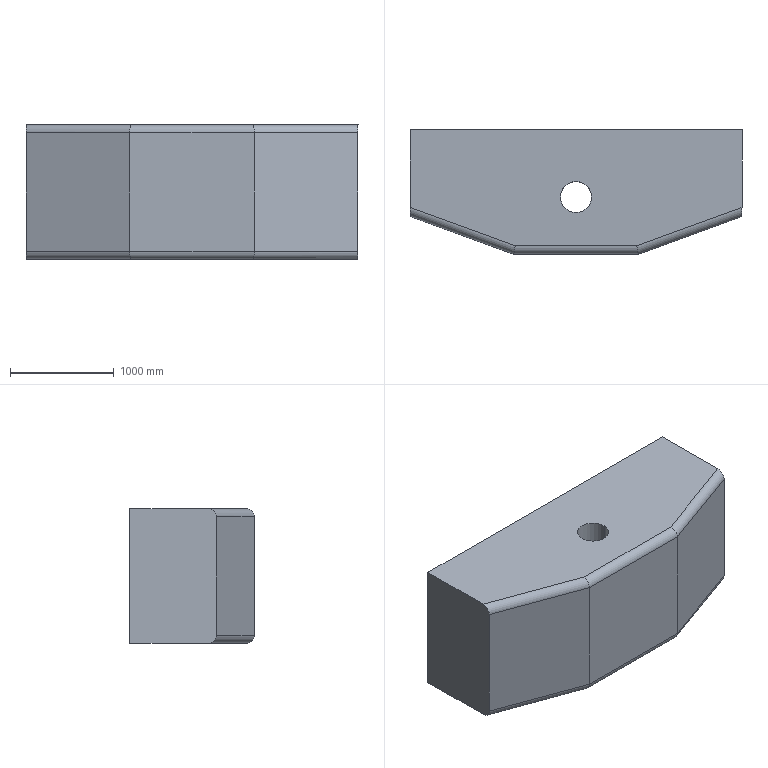Component | SolidWorks | RunningMechanism-5_7-1 | 1 solid | 16 faces | box 3200 x 1200 x 1300 mm | volume 4417803328 mm3 | cylinder 8 | plane 8 | commonest cylinder face diameters 160 x6 300 x2
build123d program:
from build123d import *

# Parameters (mm, degrees)
BOSS_EXTRUDE1_DEPTH = 650
SKETCH2_R           = 150
CUT_EXTRUDE1_DEPTH  = 2386.372
FILLET1_R           = 80


with BuildPart() as part:
    # Sketch1 → Boss-Extrude1 (new, symmetric)
    with BuildSketch(Plane.XY):
        Polygon((-1600, 0), (1600, 0), (1600, 836.03), (600, 1200), (-600, 1200), (-1600, 836.03), align=None)
    extrude(amount=BOSS_EXTRUDE1_DEPTH, both=True)

    # Sketch2 → Cut-Extrude1 (cut, through all)
    with BuildSketch(Plane.XY.offset(650)):
        with Locations((0, 650)):
            Circle(SKETCH2_R)
    extrude(amount=-CUT_EXTRUDE1_DEPTH, mode=Mode.SUBTRACT)

    # Fillet1
    fillet1_edges = [part.edges().sort_by_distance(p)[0] for p in [
        (1100, 1018.015, 650),
        (0, 1200, 650),
        (-1100, 1018.015, 650),
        (0, 1200, -650),
        (1100, 1018.015, -650),
        (-1100, 1018.015, -650),
    ]]
    fillet(fillet1_edges, radius=FILLET1_R)


solid = part.part

# Placed as in the assembly
solid = solid.moved(Location((8341.033, 54548.441, -12026.998), (180, 0, 0)))
STEP:
#1=COLOUR_RGB('',0.7922,0.8196,0.9333);
#2=FILL_AREA_STYLE_COLOUR('',#1);
#3=FILL_AREA_STYLE('',(#2));
#4=SURFACE_STYLE_FILL_AREA(#3);
#5=SURFACE_SIDE_STYLE('',(#4));
#6=SURFACE_STYLE_USAGE(.BOTH.,#5);
#7=PRESENTATION_STYLE_ASSIGNMENT((#6));
#8=CARTESIAN_POINT('',(334.293,2121.986,-499.094));
#9=VERTEX_POINT('',#8);
#10=CARTESIAN_POINT('',(322.482,2121.986,-499.094));
#11=VERTEX_POINT('',#10);
#12=CARTESIAN_POINT('',(328.387,2121.986,-499.094));
#13=DIRECTION('',(0.0000002,0.,1.));
#14=DIRECTION('',(-1.,0.,0.0000002));
#15=AXIS2_PLACEMENT_3D('',#12,#13,#14);
#16=CIRCLE('',#15,5.906);
#17=EDGE_CURVE('',#9,#11,#16,.T.);
#18=ORIENTED_EDGE('',*,*,#17,.F.);
#19=CARTESIAN_POINT('',(334.293,2121.986,-447.913));
#20=VERTEX_POINT('',#19);
#21=CARTESIAN_POINT('',(334.293,2121.986,-499.094));
#22=DIRECTION('',(0.0000002,0.,1.));
#23=VECTOR('',#22,39.37);
#24=LINE('',#21,#23);
#25=EDGE_CURVE('',#9,#20,#24,.T.);
#26=ORIENTED_EDGE('',*,*,#25,.T.);
#27=CARTESIAN_POINT('',(322.482,2121.986,-447.913));
#28=VERTEX_POINT('',#27);
#29=CARTESIAN_POINT('',(328.387,2121.986,-447.913));
#30=DIRECTION('',(0.0000002,0.,1.));
#31=DIRECTION('',(-1.,0.,0.0000002));
#32=AXIS2_PLACEMENT_3D('',#29,#30,#31);
#33=CIRCLE('',#32,5.906);
#34=EDGE_CURVE('',#20,#28,#33,.T.);
#35=ORIENTED_EDGE('',*,*,#34,.T.);
#36=CARTESIAN_POINT('',(322.482,2121.986,-499.094));
#37=DIRECTION('',(0.0000002,0.,1.));
#38=VECTOR('',#37,39.37);
#39=LINE('',#36,#38);
#40=EDGE_CURVE('',#11,#28,#39,.T.);
#41=ORIENTED_EDGE('',*,*,#40,.F.);
#42=EDGE_LOOP('',(#18,#26,#35,#41));
#43=FACE_OUTER_BOUND('',#42,.T.);
#44=CARTESIAN_POINT('',(328.387,2121.986,-499.094));
#45=DIRECTION('',(0.0000002,0.,1.));
#46=DIRECTION('',(-1.,0.,0.0000002));
#47=AXIS2_PLACEMENT_3D('',#44,#45,#46);
#48=CYLINDRICAL_SURFACE('',#47,5.906);
#49=ADVANCED_FACE('',(#43),#48,.F.);
#50=CARTESIAN_POINT('',(352.009,2100.332,-451.063));
#51=VERTEX_POINT('',#50);
#52=CARTESIAN_POINT('',(352.009,2100.332,-495.945));
#53=VERTEX_POINT('',#52);
#54=CARTESIAN_POINT('',(352.009,2100.332,-447.913));
#55=DIRECTION('',(-0.0000002,-0.,-1.));
#56=VECTOR('',#55,39.37);
#57=LINE('',#54,#56);
#58=EDGE_CURVE('',#51,#53,#57,.T.);
#59=ORIENTED_EDGE('',*,*,#58,.T.);
#60=CARTESIAN_POINT('',(391.379,2114.662,-495.945));
#61=VERTEX_POINT('',#60);
#62=CARTESIAN_POINT('',(352.009,2100.332,-495.945));
#63=DIRECTION('',(0.9397,0.342,-0.00000019));
#64=VECTOR('',#63,39.37);
#65=LINE('',#62,#64);
#66=EDGE_CURVE('',#53,#61,#65,.T.);
#67=ORIENTED_EDGE('',*,*,#66,.T.);
#68=CARTESIAN_POINT('',(391.379,2114.662,-451.063));
#69=VERTEX_POINT('',#68);
#70=CARTESIAN_POINT('',(391.379,2114.662,-447.913));
#71=DIRECTION('',(-0.0000002,-0.,-1.));
#72=VECTOR('',#71,39.37);
#73=LINE('',#70,#72);
#74=EDGE_CURVE('',#69,#61,#73,.T.);
#75=ORIENTED_EDGE('',*,*,#74,.F.);
#76=CARTESIAN_POINT('',(352.009,2100.332,-451.063));
#77=DIRECTION('',(-0.9397,-0.342,0.00000019));
#78=VECTOR('',#77,39.37);
#79=LINE('',#76,#78);
#80=EDGE_CURVE('',#69,#51,#79,.T.);
#81=ORIENTED_EDGE('',*,*,#80,.T.);
#82=EDGE_LOOP('',(#59,#67,#75,#81));
#83=FACE_OUTER_BOUND('',#82,.T.);
#84=CARTESIAN_POINT('',(352.009,2100.332,-447.913));
#85=DIRECTION('',(-0.342,0.9397,0.00000007));
#86=DIRECTION('',(-0.9397,-0.342,0.00000019));
#87=AXIS2_PLACEMENT_3D('',#84,#85,#86);
#88=PLANE('',#87);
#89=ADVANCED_FACE('',(#83),#88,.F.);
#90=ORIENTED_EDGE('',*,*,#74,.T.);
#91=CARTESIAN_POINT('',(391.379,2118.014,-499.094));
#92=VERTEX_POINT('',#91);
#93=CARTESIAN_POINT('',(391.379,2114.662,-495.945));
#94=CARTESIAN_POINT('',(391.379,2114.662,-497.79));
#95=CARTESIAN_POINT('',(391.379,2116.05,-499.094));
#96=CARTESIAN_POINT('',(391.379,2118.014,-499.094));
#97=(BOUNDED_CURVE()B_SPLINE_CURVE(3,(#93,#94,#95,#96),.UNSPECIFIED.,.F.,.T.)B_SPLINE_CURVE_WITH_KNOTS((4,4),(3.142,4.712),.UNSPECIFIED.)CURVE()GEOMETRIC_REPRESENTATION_ITEM()RATIONAL_B_SPLINE_CURVE((1.,0.8047,0.8047,1.))REPRESENTATION_ITEM(''));
#98=EDGE_CURVE('',#61,#92,#97,.T.);
#99=ORIENTED_EDGE('',*,*,#98,.T.);
#100=CARTESIAN_POINT('',(391.379,2147.576,-499.094));
#101=VERTEX_POINT('',#100);
#102=CARTESIAN_POINT('',(391.379,2114.662,-499.094));
#103=DIRECTION('',(-0.,1.,-0.));
#104=VECTOR('',#103,39.37);
#105=LINE('',#102,#104);
#106=EDGE_CURVE('',#92,#101,#105,.T.);
#107=ORIENTED_EDGE('',*,*,#106,.T.);
#108=CARTESIAN_POINT('',(391.379,2147.576,-447.913));
#109=VERTEX_POINT('',#108);
#110=CARTESIAN_POINT('',(391.379,2147.576,-447.913));
#111=DIRECTION('',(-0.0000002,-0.,-1.));
#112=VECTOR('',#111,39.37);
#113=LINE('',#110,#112);
#114=EDGE_CURVE('',#109,#101,#113,.T.);
#115=ORIENTED_EDGE('',*,*,#114,.F.);
#116=CARTESIAN_POINT('',(391.379,2118.014,-447.913));
#117=VERTEX_POINT('',#116);
#118=CARTESIAN_POINT('',(391.379,2114.662,-447.913));
#119=DIRECTION('',(-0.,1.,-0.));
#120=VECTOR('',#119,39.37);
#121=LINE('',#118,#120);
#122=EDGE_CURVE('',#117,#109,#121,.T.);
#123=ORIENTED_EDGE('',*,*,#122,.F.);
#124=CARTESIAN_POINT('',(391.379,2118.014,-447.913));
#125=CARTESIAN_POINT('',(391.379,2116.05,-447.913));
#126=CARTESIAN_POINT('',(391.379,2114.662,-449.218));
#127=CARTESIAN_POINT('',(391.379,2114.662,-451.063));
#128=(BOUNDED_CURVE()B_SPLINE_CURVE(3,(#124,#125,#126,#127),.UNSPECIFIED.,.F.,.T.)B_SPLINE_CURVE_WITH_KNOTS((4,4),(4.712,6.283),.UNSPECIFIED.)CURVE()GEOMETRIC_REPRESENTATION_ITEM()RATIONAL_B_SPLINE_CURVE((1.,0.8047,0.8047,1.))REPRESENTATION_ITEM(''));
#129=EDGE_CURVE('',#117,#69,#128,.T.);
#130=ORIENTED_EDGE('',*,*,#129,.T.);
#131=EDGE_LOOP('',(#90,#99,#107,#115,#123,#130));
#132=FACE_OUTER_BOUND('',#131,.T.);
#133=CARTESIAN_POINT('',(391.379,2114.662,-447.913));
#134=DIRECTION('',(-1.,-0.,0.0000002));
#135=DIRECTION('',(0.,-1.,0.));
#136=AXIS2_PLACEMENT_3D('',#133,#134,#135);
#137=PLANE('',#136);
#138=ADVANCED_FACE('',(#132),#137,.F.);
#139=CARTESIAN_POINT('',(265.395,2147.576,-499.094));
#140=VERTEX_POINT('',#139);
#141=CARTESIAN_POINT('',(391.379,2147.576,-499.094));
#142=DIRECTION('',(-1.,0.,0.0000002));
#143=VECTOR('',#142,39.37);
#144=LINE('',#141,#143);
#145=EDGE_CURVE('',#101,#140,#144,.T.);
#146=ORIENTED_EDGE('',*,*,#145,.T.);
#147=CARTESIAN_POINT('',(265.395,2147.576,-447.913));
#148=VERTEX_POINT('',#147);
#149=CARTESIAN_POINT('',(265.395,2147.576,-447.913));
#150=DIRECTION('',(-0.0000002,-0.,-1.));
#151=VECTOR('',#150,39.37);
#152=LINE('',#149,#151);
#153=EDGE_CURVE('',#148,#140,#152,.T.);
#154=ORIENTED_EDGE('',*,*,#153,.F.);
#155=CARTESIAN_POINT('',(391.379,2147.576,-447.913));
#156=DIRECTION('',(-1.,0.,0.0000002));
#157=VECTOR('',#156,39.37);
#158=LINE('',#155,#157);
#159=EDGE_CURVE('',#109,#148,#158,.T.);
#160=ORIENTED_EDGE('',*,*,#159,.F.);
#161=ORIENTED_EDGE('',*,*,#114,.T.);
#162=EDGE_LOOP('',(#146,#154,#160,#161));
#163=FACE_OUTER_BOUND('',#162,.T.);
#164=CARTESIAN_POINT('',(391.379,2147.576,-447.913));
#165=DIRECTION('',(-0.,-1.,0.));
#166=DIRECTION('',(1.,-0.,-0.0000002));
#167=AXIS2_PLACEMENT_3D('',#164,#165,#166);
#168=PLANE('',#167);
#169=ADVANCED_FACE('',(#163),#168,.F.);
#170=CARTESIAN_POINT('',(265.395,2118.014,-499.094));
#171=VERTEX_POINT('',#170);
#172=CARTESIAN_POINT('',(265.395,2114.662,-499.094));
#173=DIRECTION('',(-0.,-1.,0.));
#174=VECTOR('',#173,39.37);
#175=LINE('',#172,#174);
#176=EDGE_CURVE('',#140,#171,#175,.T.);
#177=ORIENTED_EDGE('',*,*,#176,.T.);
#178=CARTESIAN_POINT('',(265.395,2114.662,-495.945));
#179=VERTEX_POINT('',#178);
#180=CARTESIAN_POINT('',(265.395,2118.014,-499.094));
#181=CARTESIAN_POINT('',(265.395,2116.05,-499.094));
#182=CARTESIAN_POINT('',(265.395,2114.662,-497.79));
#183=CARTESIAN_POINT('',(265.395,2114.662,-495.945));
#184=(BOUNDED_CURVE()B_SPLINE_CURVE(3,(#180,#181,#182,#183),.UNSPECIFIED.,.F.,.T.)B_SPLINE_CURVE_WITH_KNOTS((4,4),(4.712,6.283),.UNSPECIFIED.)CURVE()GEOMETRIC_REPRESENTATION_ITEM()RATIONAL_B_SPLINE_CURVE((1.,0.8047,0.8047,1.))REPRESENTATION_ITEM(''));
#185=EDGE_CURVE('',#171,#179,#184,.T.);
#186=ORIENTED_EDGE('',*,*,#185,.T.);
#187=CARTESIAN_POINT('',(265.395,2114.662,-451.063));
#188=VERTEX_POINT('',#187);
#189=CARTESIAN_POINT('',(265.395,2114.662,-447.913));
#190=DIRECTION('',(-0.0000002,-0.,-1.));
#191=VECTOR('',#190,39.37);
#192=LINE('',#189,#191);
#193=EDGE_CURVE('',#188,#179,#192,.T.);
#194=ORIENTED_EDGE('',*,*,#193,.F.);
#195=CARTESIAN_POINT('',(265.395,2118.014,-447.913));
#196=VERTEX_POINT('',#195);
#197=CARTESIAN_POINT('',(265.395,2114.662,-451.063));
#198=CARTESIAN_POINT('',(265.395,2114.662,-449.218));
#199=CARTESIAN_POINT('',(265.395,2116.05,-447.913));
#200=CARTESIAN_POINT('',(265.395,2118.014,-447.913));
#201=(BOUNDED_CURVE()B_SPLINE_CURVE(3,(#197,#198,#199,#200),.UNSPECIFIED.,.F.,.F.)B_SPLINE_CURVE_WITH_KNOTS((4,4),(3.142,4.712),.UNSPECIFIED.)CURVE()GEOMETRIC_REPRESENTATION_ITEM()RATIONAL_B_SPLINE_CURVE((1.,0.8047,0.8047,1.))REPRESENTATION_ITEM(''));
#202=EDGE_CURVE('',#188,#196,#201,.T.);
#203=ORIENTED_EDGE('',*,*,#202,.T.);
#204=CARTESIAN_POINT('',(265.395,2114.662,-447.913));
#205=DIRECTION('',(-0.,-1.,0.));
#206=VECTOR('',#205,39.37);
#207=LINE('',#204,#206);
#208=EDGE_CURVE('',#148,#196,#207,.T.);
#209=ORIENTED_EDGE('',*,*,#208,.F.);
#210=ORIENTED_EDGE('',*,*,#153,.T.);
#211=EDGE_LOOP('',(#177,#186,#194,#203,#209,#210));
#212=FACE_OUTER_BOUND('',#211,.T.);
#213=CARTESIAN_POINT('',(265.395,2114.662,-447.913));
#214=DIRECTION('',(1.,-0.,-0.0000002));
#215=DIRECTION('',(0.0000002,0.,1.));
#216=AXIS2_PLACEMENT_3D('',#213,#214,#215);
#217=PLANE('',#216);
#218=ADVANCED_FACE('',(#212),#217,.F.);
#219=ORIENTED_EDGE('',*,*,#193,.T.);
#220=CARTESIAN_POINT('',(304.765,2100.332,-495.945));
#221=VERTEX_POINT('',#220);
#222=CARTESIAN_POINT('',(304.765,2100.332,-495.945));
#223=DIRECTION('',(0.9397,-0.342,-0.00000019));
#224=VECTOR('',#223,39.37);
#225=LINE('',#222,#224);
#226=EDGE_CURVE('',#179,#221,#225,.T.);
#227=ORIENTED_EDGE('',*,*,#226,.T.);
#228=CARTESIAN_POINT('',(304.765,2100.332,-451.063));
#229=VERTEX_POINT('',#228);
#230=CARTESIAN_POINT('',(304.765,2100.332,-447.913));
#231=DIRECTION('',(-0.0000002,-0.,-1.));
#232=VECTOR('',#231,39.37);
#233=LINE('',#230,#232);
#234=EDGE_CURVE('',#229,#221,#233,.T.);
#235=ORIENTED_EDGE('',*,*,#234,.F.);
#236=CARTESIAN_POINT('',(265.395,2114.662,-451.063));
#237=DIRECTION('',(-0.9397,0.342,0.00000019));
#238=VECTOR('',#237,39.37);
#239=LINE('',#236,#238);
#240=EDGE_CURVE('',#229,#188,#239,.T.);
#241=ORIENTED_EDGE('',*,*,#240,.T.);
#242=EDGE_LOOP('',(#219,#227,#235,#241));
#243=FACE_OUTER_BOUND('',#242,.T.);
#244=CARTESIAN_POINT('',(304.765,2100.332,-447.913));
#245=DIRECTION('',(0.342,0.9397,-0.00000007));
#246=DIRECTION('',(-0.9397,0.342,0.00000019));
#247=AXIS2_PLACEMENT_3D('',#244,#245,#246);
#248=PLANE('',#247);
#249=ADVANCED_FACE('',(#243),#248,.F.);
#250=ORIENTED_EDGE('',*,*,#234,.T.);
#251=CARTESIAN_POINT('',(304.765,2100.332,-495.945));
#252=DIRECTION('',(1.,0.,-0.0000002));
#253=VECTOR('',#252,39.37);
#254=LINE('',#251,#253);
#255=EDGE_CURVE('',#221,#53,#254,.T.);
#256=ORIENTED_EDGE('',*,*,#255,.T.);
#257=ORIENTED_EDGE('',*,*,#58,.F.);
#258=CARTESIAN_POINT('',(304.765,2100.332,-451.063));
#259=DIRECTION('',(-1.,-0.,0.0000002));
#260=VECTOR('',#259,39.37);
#261=LINE('',#258,#260);
#262=EDGE_CURVE('',#51,#229,#261,.T.);
#263=ORIENTED_EDGE('',*,*,#262,.T.);
#264=EDGE_LOOP('',(#250,#256,#257,#263));
#265=FACE_OUTER_BOUND('',#264,.T.);
#266=CARTESIAN_POINT('',(304.765,2100.332,-447.913));
#267=DIRECTION('',(-0.,1.,-0.));
#268=DIRECTION('',(-1.,-0.,0.0000002));
#269=AXIS2_PLACEMENT_3D('',#266,#267,#268);
#270=PLANE('',#269);
#271=ADVANCED_FACE('',(#265),#270,.F.);
#272=CARTESIAN_POINT('',(328.387,2121.986,-447.913));
#273=DIRECTION('',(0.0000002,0.,1.));
#274=DIRECTION('',(-1.,0.,0.0000002));
#275=AXIS2_PLACEMENT_3D('',#272,#273,#274);
#276=CIRCLE('',#275,5.906);
#277=EDGE_CURVE('',#28,#20,#276,.T.);
#278=ORIENTED_EDGE('',*,*,#277,.F.);
#279=ORIENTED_EDGE('',*,*,#34,.F.);
#280=EDGE_LOOP('',(#278,#279));
#281=FACE_BOUND('',#280,.T.);
#282=CARTESIAN_POINT('',(305.32,2103.482,-447.913));
#283=VERTEX_POINT('',#282);
#284=CARTESIAN_POINT('',(351.454,2103.482,-447.913));
#285=VERTEX_POINT('',#284);
#286=CARTESIAN_POINT('',(352.009,2103.482,-447.913));
#287=DIRECTION('',(1.,0.,-0.0000002));
#288=VECTOR('',#287,39.37);
#289=LINE('',#286,#288);
#290=EDGE_CURVE('',#283,#285,#289,.T.);
#291=ORIENTED_EDGE('',*,*,#290,.T.);
#292=CARTESIAN_POINT('',(390.302,2117.622,-447.913));
#293=DIRECTION('',(0.9397,0.342,-0.00000019));
#294=VECTOR('',#293,39.37);
#295=LINE('',#292,#294);
#296=EDGE_CURVE('',#285,#117,#295,.T.);
#297=ORIENTED_EDGE('',*,*,#296,.T.);
#298=ORIENTED_EDGE('',*,*,#122,.T.);
#299=ORIENTED_EDGE('',*,*,#159,.T.);
#300=ORIENTED_EDGE('',*,*,#208,.T.);
#301=CARTESIAN_POINT('',(305.842,2103.292,-447.913));
#302=DIRECTION('',(0.9397,-0.342,-0.00000019));
#303=VECTOR('',#302,39.37);
#304=LINE('',#301,#303);
#305=EDGE_CURVE('',#196,#283,#304,.T.);
#306=ORIENTED_EDGE('',*,*,#305,.T.);
#307=EDGE_LOOP('',(#291,#297,#298,#299,#300,#306));
#308=FACE_OUTER_BOUND('',#307,.T.);
#309=CARTESIAN_POINT('',(328.387,2147.576,-447.913));
#310=DIRECTION('',(0.0000002,0.,1.));
#311=DIRECTION('',(-1.,0.,0.0000002));
#312=AXIS2_PLACEMENT_3D('',#309,#310,#311);
#313=PLANE('',#312);
#314=ADVANCED_FACE('',(#281,#308),#313,.T.);
#315=CARTESIAN_POINT('',(328.387,2121.986,-499.094));
#316=DIRECTION('',(0.0000002,0.,1.));
#317=DIRECTION('',(-1.,0.,0.0000002));
#318=AXIS2_PLACEMENT_3D('',#315,#316,#317);
#319=CIRCLE('',#318,5.906);
#320=EDGE_CURVE('',#11,#9,#319,.T.);
#321=ORIENTED_EDGE('',*,*,#320,.T.);
#322=ORIENTED_EDGE('',*,*,#17,.T.);
#323=EDGE_LOOP('',(#321,#322));
#324=FACE_BOUND('',#323,.T.);
#325=CARTESIAN_POINT('',(351.454,2103.482,-499.094));
#326=VERTEX_POINT('',#325);
#327=CARTESIAN_POINT('',(305.32,2103.482,-499.094));
#328=VERTEX_POINT('',#327);
#329=CARTESIAN_POINT('',(328.387,2103.482,-499.094));
#330=DIRECTION('',(-1.,-0.,0.0000002));
#331=VECTOR('',#330,39.37);
#332=LINE('',#329,#331);
#333=EDGE_CURVE('',#326,#328,#332,.T.);
#334=ORIENTED_EDGE('',*,*,#333,.T.);
#335=CARTESIAN_POINT('',(311.517,2101.227,-499.094));
#336=DIRECTION('',(-0.9397,0.342,0.00000019));
#337=VECTOR('',#336,39.37);
#338=LINE('',#335,#337);
#339=EDGE_CURVE('',#328,#171,#338,.T.);
#340=ORIENTED_EDGE('',*,*,#339,.T.);
#341=ORIENTED_EDGE('',*,*,#176,.F.);
#342=ORIENTED_EDGE('',*,*,#145,.F.);
#343=ORIENTED_EDGE('',*,*,#106,.F.);
#344=CARTESIAN_POINT('',(345.257,2101.227,-499.094));
#345=DIRECTION('',(-0.9397,-0.342,0.00000019));
#346=VECTOR('',#345,39.37);
#347=LINE('',#344,#346);
#348=EDGE_CURVE('',#92,#326,#347,.T.);
#349=ORIENTED_EDGE('',*,*,#348,.T.);
#350=EDGE_LOOP('',(#334,#340,#341,#342,#343,#349));
#351=FACE_OUTER_BOUND('',#350,.T.);
#352=CARTESIAN_POINT('',(328.387,2147.576,-499.094));
#353=DIRECTION('',(0.0000002,0.,1.));
#354=DIRECTION('',(-1.,0.,0.0000002));
#355=AXIS2_PLACEMENT_3D('',#352,#353,#354);
#356=PLANE('',#355);
#357=ADVANCED_FACE('',(#324,#351),#356,.F.);
#358=ORIENTED_EDGE('',*,*,#25,.F.);
#359=ORIENTED_EDGE('',*,*,#320,.F.);
#360=ORIENTED_EDGE('',*,*,#40,.T.);
#361=ORIENTED_EDGE('',*,*,#277,.T.);
#362=EDGE_LOOP('',(#358,#359,#360,#361));
#363=FACE_OUTER_BOUND('',#362,.T.);
#364=CARTESIAN_POINT('',(328.387,2121.986,-499.094));
#365=DIRECTION('',(0.0000002,0.,1.));
#366=DIRECTION('',(-1.,0.,0.0000002));
#367=AXIS2_PLACEMENT_3D('',#364,#365,#366);
#368=CYLINDRICAL_SURFACE('',#367,5.906);
#369=ADVANCED_FACE('',(#363),#368,.F.);
#370=ORIENTED_EDGE('',*,*,#98,.F.);
#371=ORIENTED_EDGE('',*,*,#66,.F.);
#372=CARTESIAN_POINT('',(351.454,2103.482,-499.094));
#373=CARTESIAN_POINT('',(351.779,2101.637,-499.094));
#374=CARTESIAN_POINT('',(352.009,2100.332,-497.79));
#375=CARTESIAN_POINT('',(352.009,2100.332,-495.945));
#376=(BOUNDED_CURVE()B_SPLINE_CURVE(3,(#372,#373,#374,#375),.UNSPECIFIED.,.F.,.T.)B_SPLINE_CURVE_WITH_KNOTS((4,4),(1.571,3.142),.UNSPECIFIED.)CURVE()GEOMETRIC_REPRESENTATION_ITEM()RATIONAL_B_SPLINE_CURVE((1.,0.8047,0.8047,1.))REPRESENTATION_ITEM(''));
#377=EDGE_CURVE('',#326,#53,#376,.T.);
#378=ORIENTED_EDGE('',*,*,#377,.F.);
#379=ORIENTED_EDGE('',*,*,#348,.F.);
#380=EDGE_LOOP('',(#370,#371,#378,#379));
#381=FACE_OUTER_BOUND('',#380,.T.);
#382=CARTESIAN_POINT('',(350.932,2103.292,-495.945));
#383=DIRECTION('',(0.9397,0.342,-0.00000019));
#384=DIRECTION('',(-0.342,0.9397,0.00000007));
#385=AXIS2_PLACEMENT_3D('',#382,#383,#384);
#386=CYLINDRICAL_SURFACE('',#385,3.15);
#387=ADVANCED_FACE('',(#381),#386,.T.);
#388=ORIENTED_EDGE('',*,*,#377,.T.);
#389=ORIENTED_EDGE('',*,*,#255,.F.);
#390=CARTESIAN_POINT('',(305.32,2103.482,-499.094));
#391=CARTESIAN_POINT('',(304.995,2101.637,-499.094));
#392=CARTESIAN_POINT('',(304.765,2100.332,-497.79));
#393=CARTESIAN_POINT('',(304.765,2100.332,-495.945));
#394=(BOUNDED_CURVE()B_SPLINE_CURVE(3,(#390,#391,#392,#393),.UNSPECIFIED.,.F.,.F.)B_SPLINE_CURVE_WITH_KNOTS((4,4),(1.571,3.142),.UNSPECIFIED.)CURVE()GEOMETRIC_REPRESENTATION_ITEM()RATIONAL_B_SPLINE_CURVE((1.,0.8047,0.8047,1.))REPRESENTATION_ITEM(''));
#395=EDGE_CURVE('',#328,#221,#394,.T.);
#396=ORIENTED_EDGE('',*,*,#395,.F.);
#397=ORIENTED_EDGE('',*,*,#333,.F.);
#398=EDGE_LOOP('',(#388,#389,#396,#397));
#399=FACE_OUTER_BOUND('',#398,.T.);
#400=CARTESIAN_POINT('',(304.765,2103.482,-495.945));
#401=DIRECTION('',(1.,0.,-0.0000002));
#402=DIRECTION('',(0.,1.,0.));
#403=AXIS2_PLACEMENT_3D('',#400,#401,#402);
#404=CYLINDRICAL_SURFACE('',#403,3.15);
#405=ADVANCED_FACE('',(#399),#404,.T.);
#406=ORIENTED_EDGE('',*,*,#185,.F.);
#407=ORIENTED_EDGE('',*,*,#339,.F.);
#408=ORIENTED_EDGE('',*,*,#395,.T.);
#409=ORIENTED_EDGE('',*,*,#226,.F.);
#410=EDGE_LOOP('',(#406,#407,#408,#409));
#411=FACE_OUTER_BOUND('',#410,.T.);
#412=CARTESIAN_POINT('',(305.842,2103.292,-495.945));
#413=DIRECTION('',(0.9397,-0.342,-0.00000019));
#414=DIRECTION('',(0.342,0.9397,-0.00000007));
#415=AXIS2_PLACEMENT_3D('',#412,#413,#414);
#416=CYLINDRICAL_SURFACE('',#415,3.15);
#417=ADVANCED_FACE('',(#411),#416,.T.);
#418=ORIENTED_EDGE('',*,*,#202,.F.);
#419=ORIENTED_EDGE('',*,*,#240,.F.);
#420=CARTESIAN_POINT('',(305.32,2103.482,-447.913));
#421=CARTESIAN_POINT('',(304.995,2101.637,-447.913));
#422=CARTESIAN_POINT('',(304.765,2100.332,-449.218));
#423=CARTESIAN_POINT('',(304.765,2100.332,-451.063));
#424=(BOUNDED_CURVE()B_SPLINE_CURVE(3,(#420,#421,#422,#423),.UNSPECIFIED.,.F.,.T.)B_SPLINE_CURVE_WITH_KNOTS((4,4),(4.712,6.283),.UNSPECIFIED.)CURVE()GEOMETRIC_REPRESENTATION_ITEM()RATIONAL_B_SPLINE_CURVE((1.,0.8047,0.8047,1.))REPRESENTATION_ITEM(''));
#425=EDGE_CURVE('',#283,#229,#424,.T.);
#426=ORIENTED_EDGE('',*,*,#425,.F.);
#427=ORIENTED_EDGE('',*,*,#305,.F.);
#428=EDGE_LOOP('',(#418,#419,#426,#427));
#429=FACE_OUTER_BOUND('',#428,.T.);
#430=CARTESIAN_POINT('',(311.517,2101.227,-451.063));
#431=DIRECTION('',(-0.9397,0.342,0.00000019));
#432=DIRECTION('',(-0.342,-0.9397,0.00000007));
#433=AXIS2_PLACEMENT_3D('',#430,#431,#432);
#434=CYLINDRICAL_SURFACE('',#433,3.15);
#435=ADVANCED_FACE('',(#429),#434,.T.);
#436=ORIENTED_EDGE('',*,*,#425,.T.);
#437=ORIENTED_EDGE('',*,*,#262,.F.);
#438=CARTESIAN_POINT('',(351.454,2103.482,-447.913));
#439=CARTESIAN_POINT('',(351.779,2101.637,-447.913));
#440=CARTESIAN_POINT('',(352.009,2100.332,-449.218));
#441=CARTESIAN_POINT('',(352.009,2100.332,-451.063));
#442=(BOUNDED_CURVE()B_SPLINE_CURVE(3,(#438,#439,#440,#441),.UNSPECIFIED.,.F.,.T.)B_SPLINE_CURVE_WITH_KNOTS((4,4),(1.571,3.142),.UNSPECIFIED.)CURVE()GEOMETRIC_REPRESENTATION_ITEM()RATIONAL_B_SPLINE_CURVE((1.,0.8047,0.8047,1.))REPRESENTATION_ITEM(''));
#443=EDGE_CURVE('',#285,#51,#442,.T.);
#444=ORIENTED_EDGE('',*,*,#443,.F.);
#445=ORIENTED_EDGE('',*,*,#290,.F.);
#446=EDGE_LOOP('',(#436,#437,#444,#445));
#447=FACE_OUTER_BOUND('',#446,.T.);
#448=CARTESIAN_POINT('',(328.387,2103.482,-451.063));
#449=DIRECTION('',(-1.,-0.,0.0000002));
#450=DIRECTION('',(0.,-1.,0.));
#451=AXIS2_PLACEMENT_3D('',#448,#449,#450);
#452=CYLINDRICAL_SURFACE('',#451,3.15);
#453=ADVANCED_FACE('',(#447),#452,.T.);
#454=ORIENTED_EDGE('',*,*,#443,.T.);
#455=ORIENTED_EDGE('',*,*,#80,.F.);
#456=ORIENTED_EDGE('',*,*,#129,.F.);
#457=ORIENTED_EDGE('',*,*,#296,.F.);
#458=EDGE_LOOP('',(#454,#455,#456,#457));
#459=FACE_OUTER_BOUND('',#458,.T.);
#460=CARTESIAN_POINT('',(345.257,2101.227,-451.063));
#461=DIRECTION('',(-0.9397,-0.342,0.00000019));
#462=DIRECTION('',(0.342,-0.9397,-0.00000007));
#463=AXIS2_PLACEMENT_3D('',#460,#461,#462);
#464=CYLINDRICAL_SURFACE('',#463,3.15);
#465=ADVANCED_FACE('',(#459),#464,.T.);
#466=CLOSED_SHELL('',(#49,#89,#138,#169,#218,#249,#271,#314,#357,#369,#387,#405,#417,#435,#453,#465));
#467=MANIFOLD_SOLID_BREP('',#466);
#468=STYLED_ITEM('',(#7),#467);
#469=PRESENTATION_LAYER_ASSIGNMENT('','',(#468));
#470=CARTESIAN_POINT('',(0.,0.,0.));
#471=DIRECTION('',(0.,0.,1.));
#472=DIRECTION('',(1.,0.,0.));
#473=AXIS2_PLACEMENT_3D('',#470,#471,#472);
#474=(LENGTH_UNIT()NAMED_UNIT(*)SI_UNIT($,.METRE.));
#475=LENGTH_MEASURE_WITH_UNIT(LENGTH_MEASURE(0.0254),#474);
#476=DIMENSIONAL_EXPONENTS(1.,0.,0.,0.,0.,0.,0.);
#477=(CONVERSION_BASED_UNIT('',#475)LENGTH_UNIT()NAMED_UNIT(#476));
#478=UNCERTAINTY_MEASURE_WITH_UNIT(LENGTH_MEASURE(0.00001),#477,'','');
#479=(NAMED_UNIT(*)PLANE_ANGLE_UNIT()SI_UNIT($,.RADIAN.));
#480=(NAMED_UNIT(*)SI_UNIT($,.STERADIAN.)SOLID_ANGLE_UNIT());
#481=(GEOMETRIC_REPRESENTATION_CONTEXT(3)GLOBAL_UNCERTAINTY_ASSIGNED_CONTEXT((#478))GLOBAL_UNIT_ASSIGNED_CONTEXT((#477,#479,#480))REPRESENTATION_CONTEXT('',''));
#482=ADVANCED_BREP_SHAPE_REPRESENTATION('',(#467,#473),#481);
#483=(LENGTH_UNIT()NAMED_UNIT(*)SI_UNIT($,.METRE.));
#484=LENGTH_MEASURE_WITH_UNIT(LENGTH_MEASURE(0.0254),#483);
#485=DIMENSIONAL_EXPONENTS(1.,0.,0.,0.,0.,0.,0.);
#486=(CONVERSION_BASED_UNIT('',#484)LENGTH_UNIT()NAMED_UNIT(#485));
#487=UNCERTAINTY_MEASURE_WITH_UNIT(LENGTH_MEASURE(0.00001),#486,'','');
#488=(NAMED_UNIT(*)PLANE_ANGLE_UNIT()SI_UNIT($,.RADIAN.));
#489=(NAMED_UNIT(*)SI_UNIT($,.STERADIAN.)SOLID_ANGLE_UNIT());
#490=(GEOMETRIC_REPRESENTATION_CONTEXT(3)GLOBAL_UNCERTAINTY_ASSIGNED_CONTEXT((#487))GLOBAL_UNIT_ASSIGNED_CONTEXT((#486,#488,#489))REPRESENTATION_CONTEXT('',''));
#491=MECHANICAL_DESIGN_GEOMETRIC_PRESENTATION_REPRESENTATION('',(#468),#490);